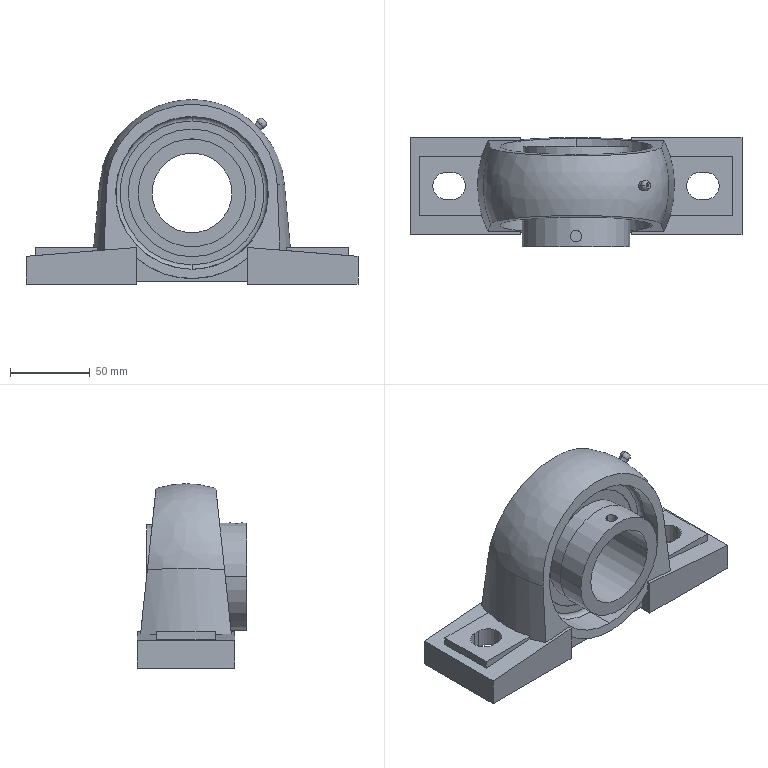Component | SolidWorks | LowerTensioningDeviceAssembly-1_GB_T7810-1995BearingWithVerticalSeatUELP210-2 | 1 solid | 124 faces | volume 432979 mm3 | plane 59 | cylinder 30 | cone 16 | sphere 8 | torus 8 | spline 3 | commonest cylinder face diameters 95.677 x6 80.04 x6 66 x6 17 x4 7.134 x2 67.6 x2 50 x2 107.263 x2